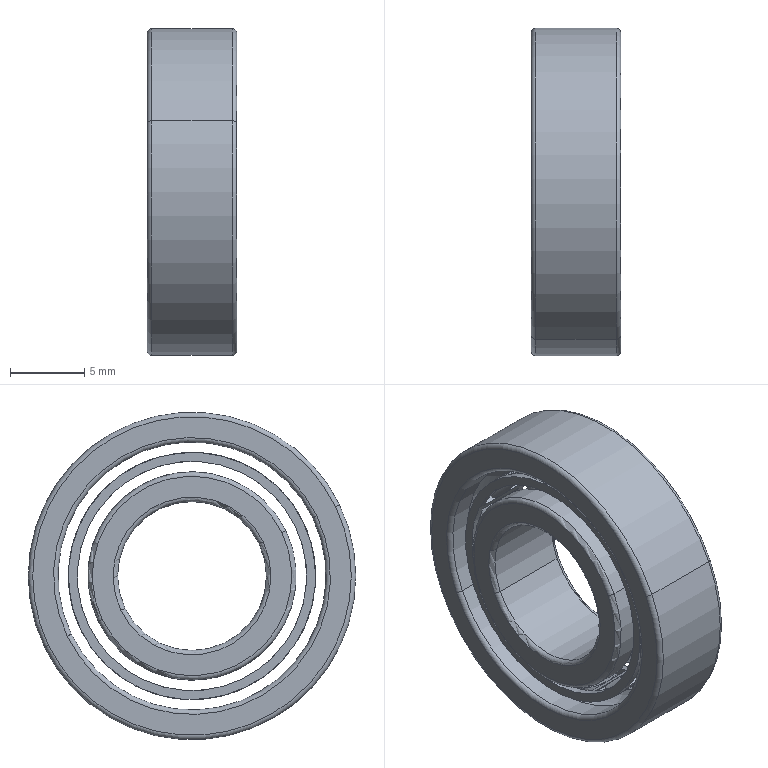Component | SolidWorks | FrontGuideWheel-1_DeepGrooveBallBearing[60000][61900]-1 | 16 solids | 152 faces | volume 1188 mm3 | cylinder 72 | plane 32 | sphere 26 | torus 22 | commonest cylinder face diameters 3.4 x28 16.6 x16 15.4 x16 18 x4 14 x4 22 x2 10 x2 | material AISI 304